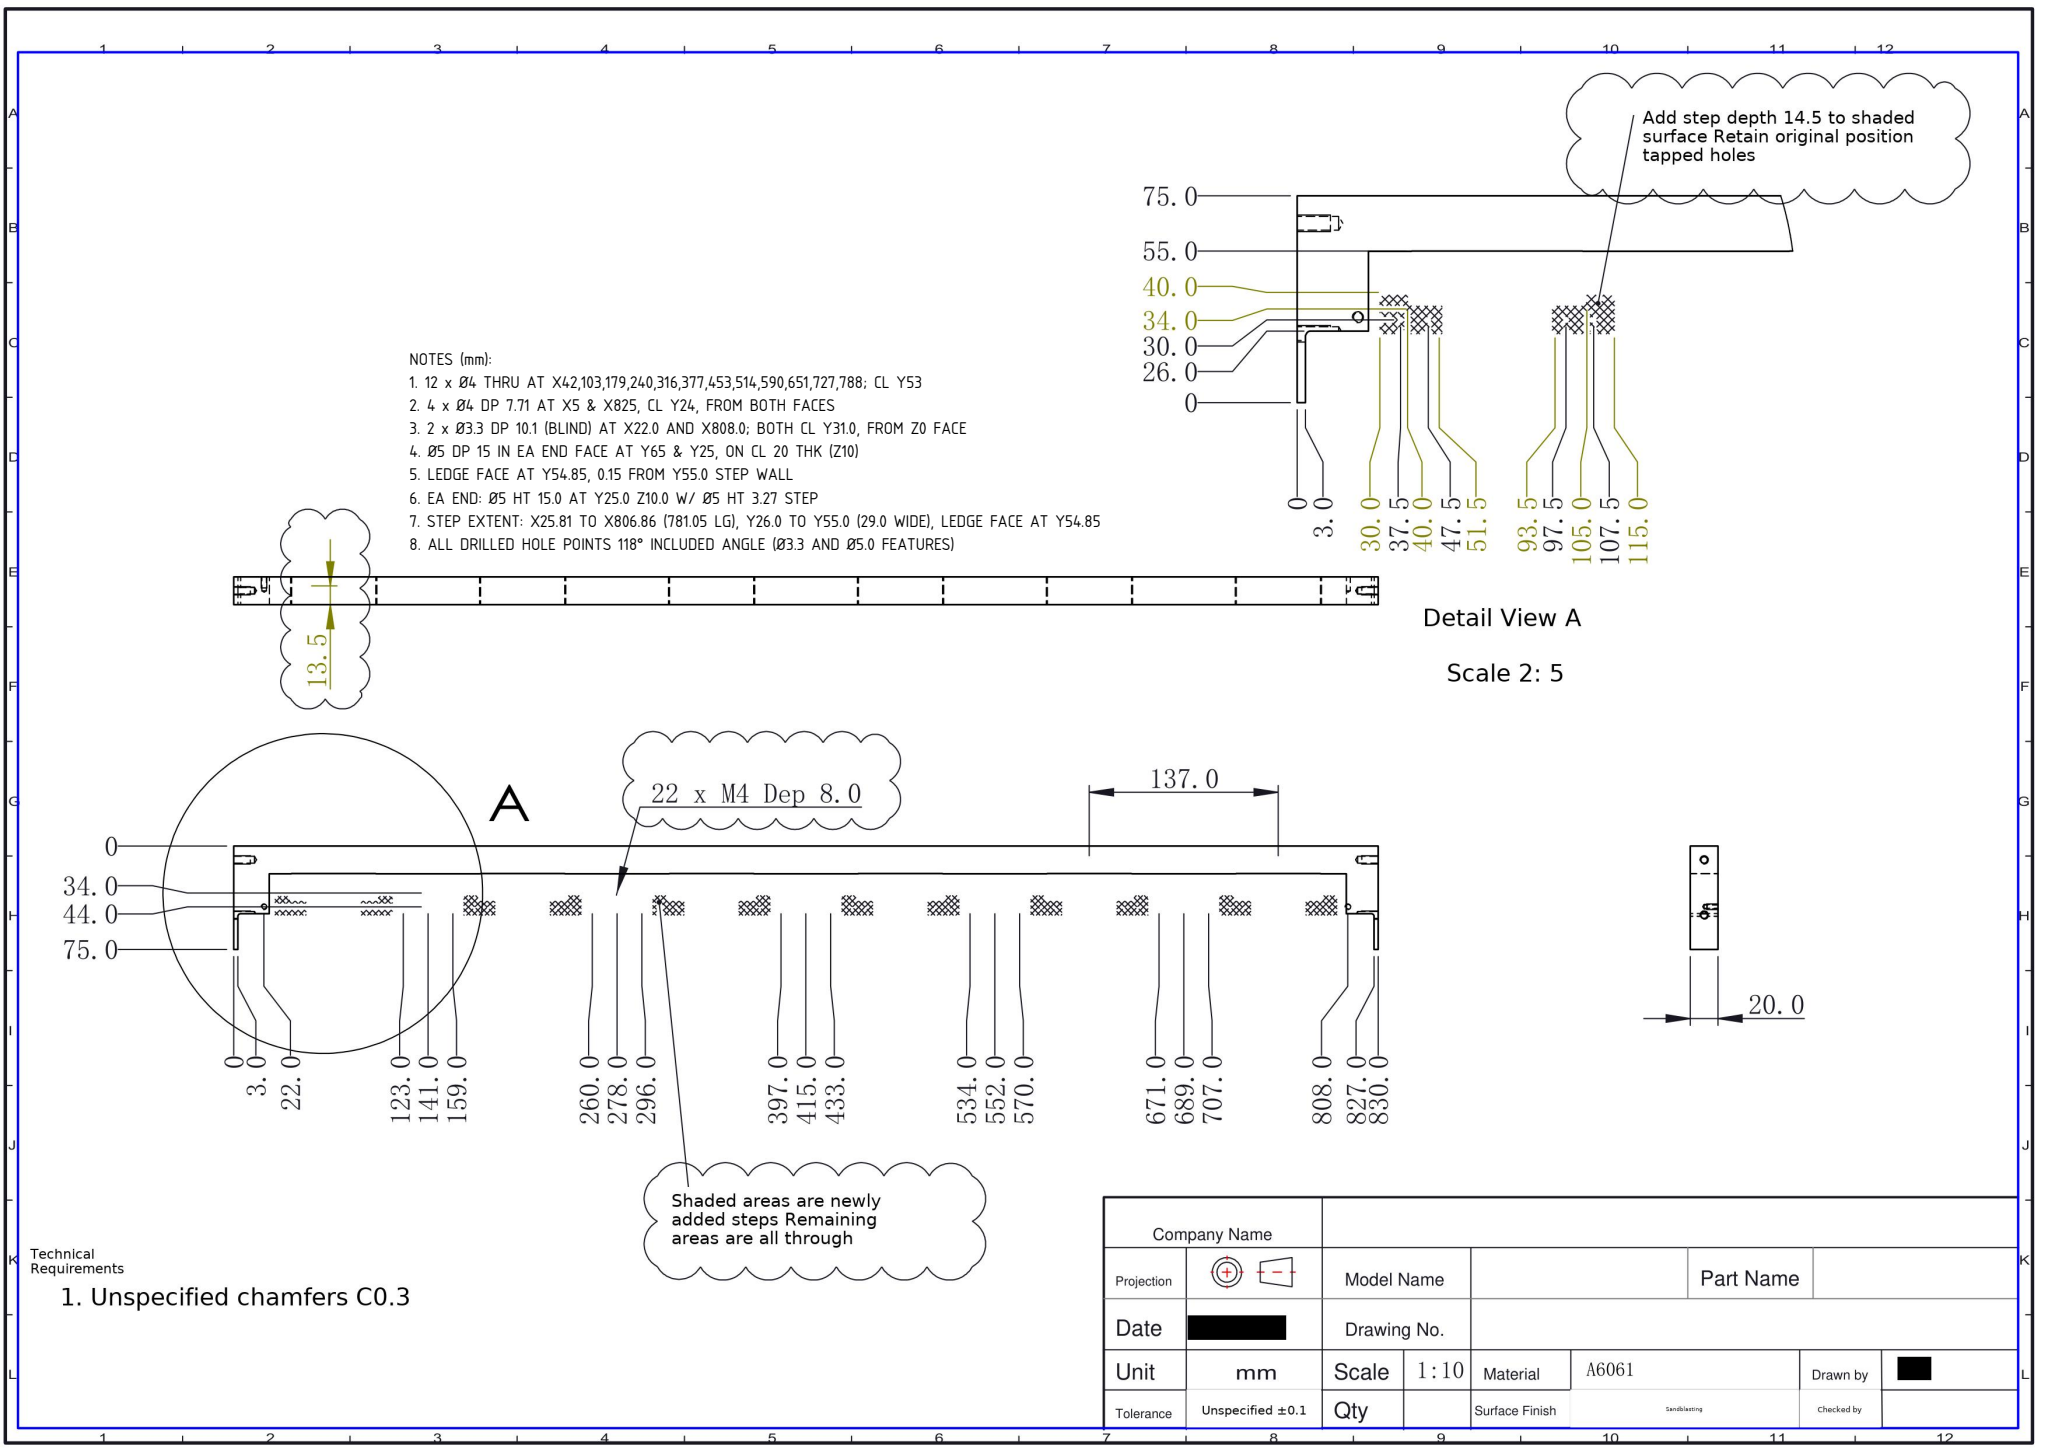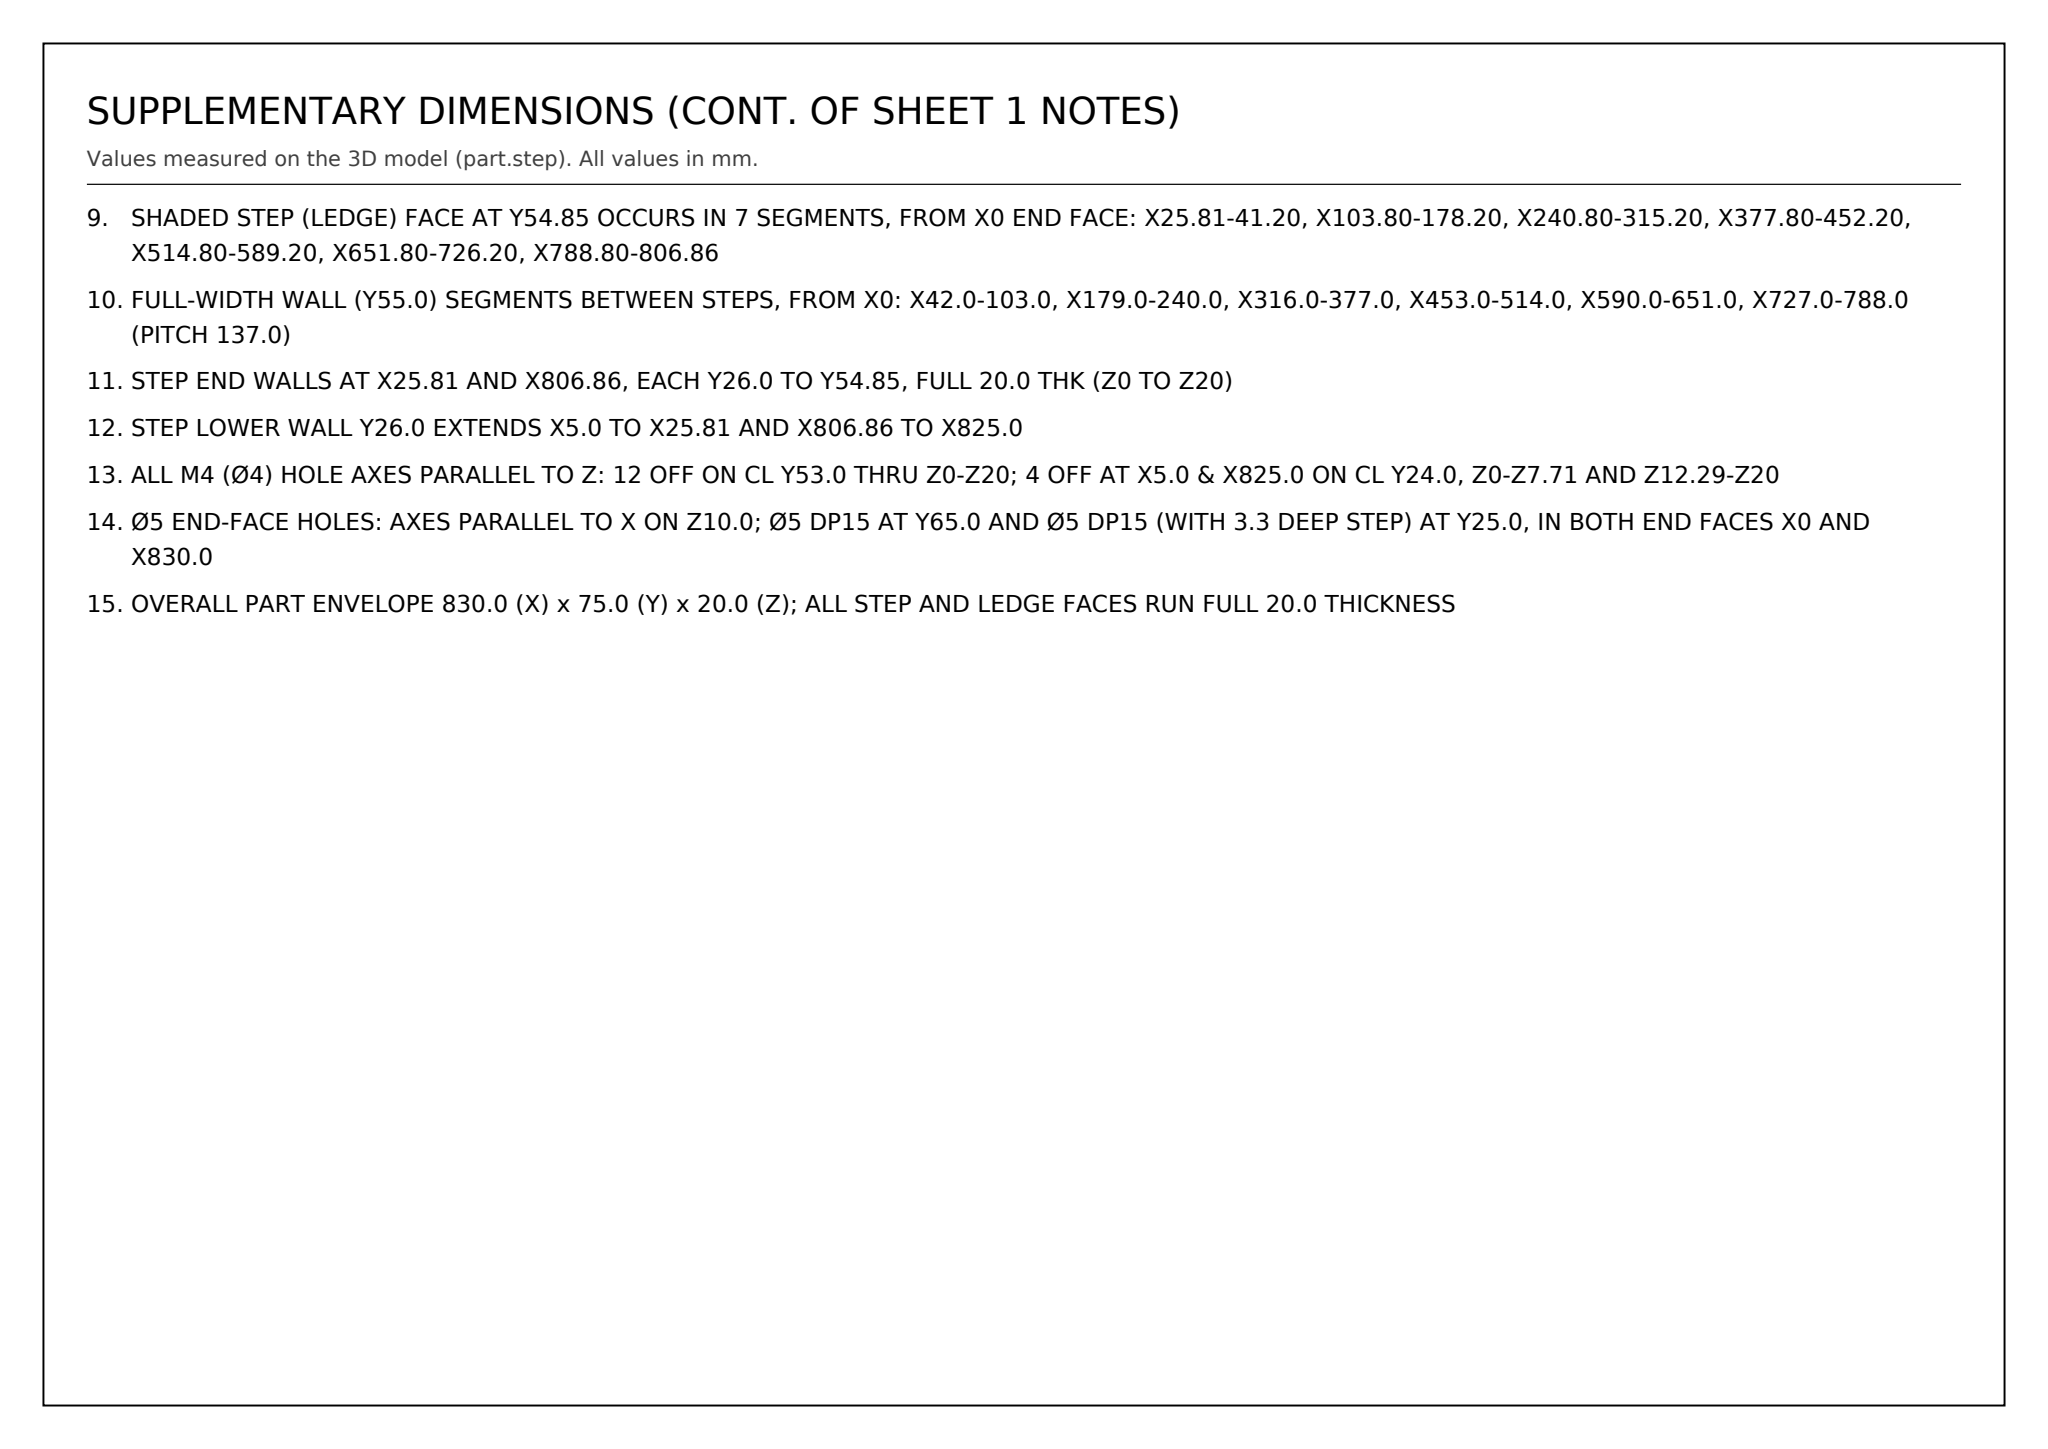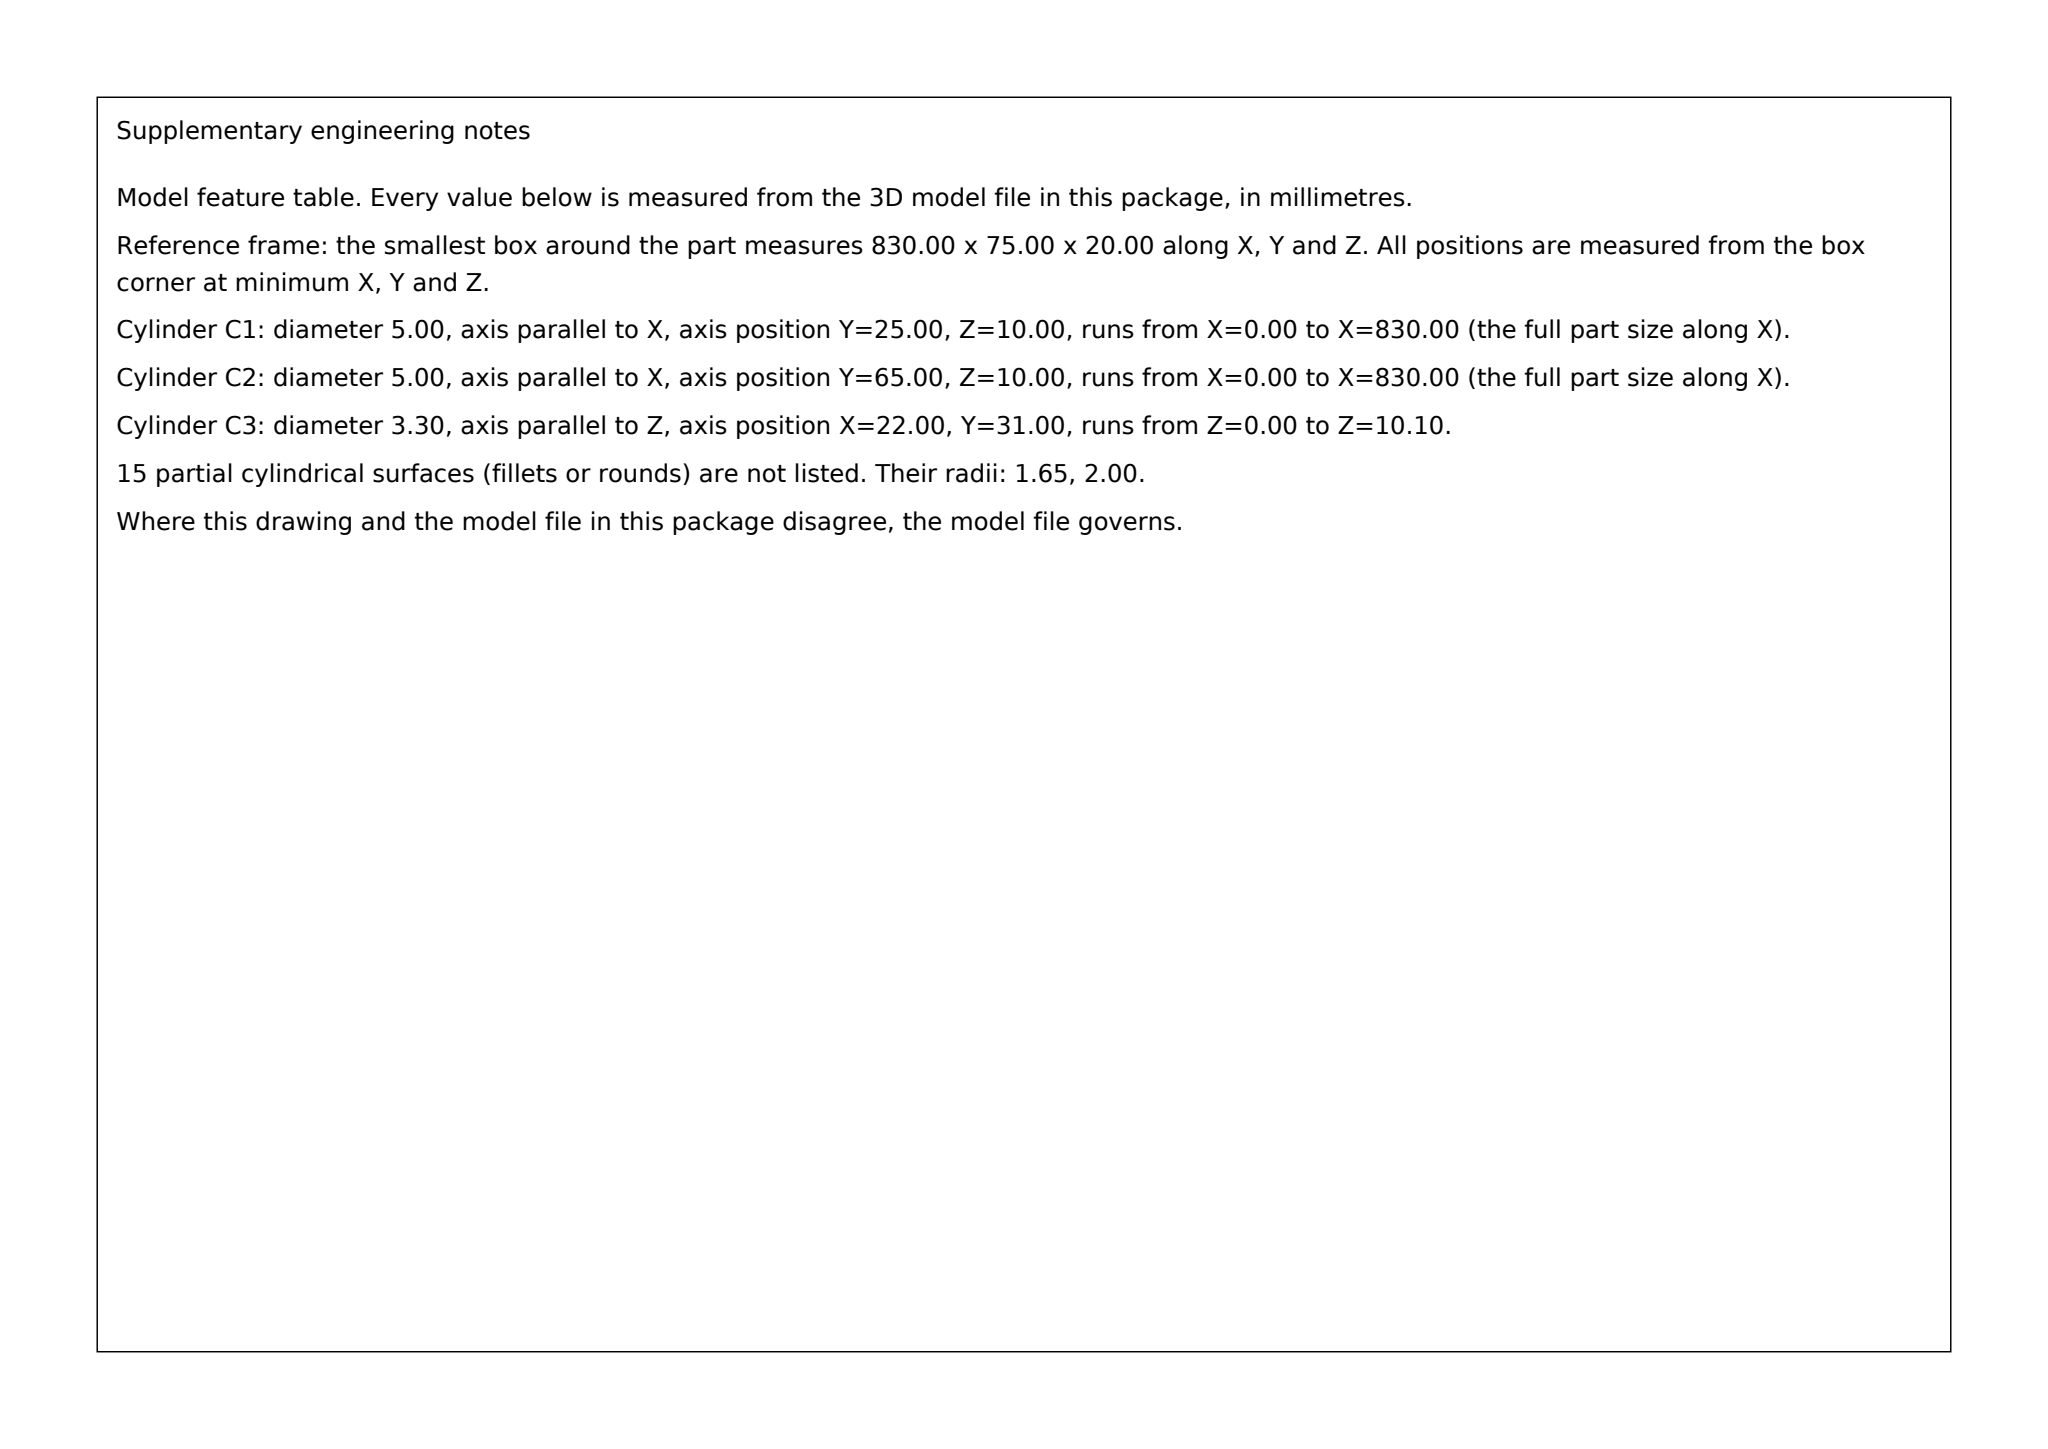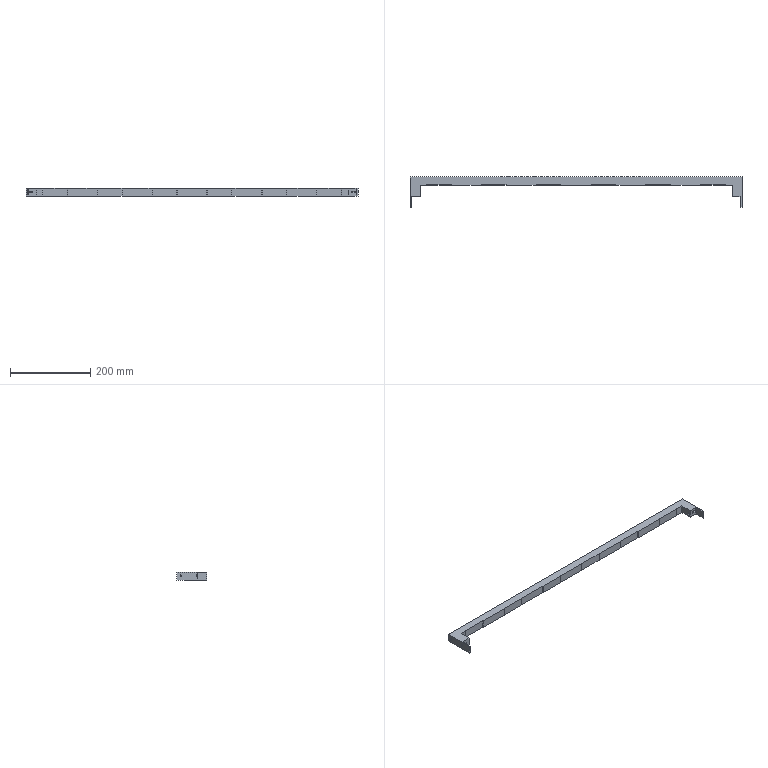Part | SolidWorks | mm | 1 solid | 63 faces | box 830 x 75 x 20 mm | volume 363775 mm3 | cylinder 27 | plane 26 | cone 10 | commonest cylinder face diameters 4 x16 5 x8 3.3 x3
Drawing notes:
12 x Ø4 THRU AT X42,103,179,240,316,377,453,514,590,651,727,788; CL Y53 | from the solid: Ø4.0 z-axis cyls L=20.0 (= full 20 thk) at y=53.0, those 12 X positions
4 x Ø4 DP 7.71 AT X5 & X825, CL Y24, FROM BOTH FACES | from the solid: Ø4.0 z-axis cyls L=7.71, count 2 each at [5,24] and [825,24]; 7.71+7.71<20 thk
2 x Ø3.3 DP 10.1 (BLIND) AT X22.0 AND X808.0; BOTH CL Y31.0, FROM Z0 FACE | from the solid: cylinders: hole/bore Ø3.3 axis z at [22.0, 31.0] from 0.0 to 10.1 (360°); Ø3.3 axis z at [808.0, 31.0] from 0.0 to 10.1 (267° arc); 118° drill-point cones at z=10.1 (bbox_from [20.4,31.0,10.1] and [806.4,31.0,10.1]); part thickness z 0-20 so holes are not through
Ø5 DP 15 IN EA END FACE AT Y65 & Y25, ON CL 20 THK (Z10) | from the solid: Ø5 x-axis cyls L=15 at [y65,z10] x4 and [y25,z10] x2; 75-65=10 from top, z10=mid-thk
LEDGE FACE AT Y54.85, 0.15 FROM Y55.0 STEP WALL | from the solid: axis_planes y=54.85 (7 faces) adjacent to y=55.0 (6 faces)
EA END: Ø5 HT 15.0 AT Y25.0 Z10.0 W/ Ø5 HT 3.27 STEP | from the solid: x-axis cyls dia 5.0 at [y25.0,z10.0]: len 15.0 count 2 and len 3.27 count 2 (one each end)
STEP EXTENT: X25.81 TO X806.86 (781.05 LG), Y26.0 TO Y55.0 (29.0 WIDE), LEDGE FACE AT Y54.85 | from the solid: axis planes x=25.81, x=806.86; y=26.0, y=54.85, y=55.0
ALL DRILLED HOLE POINTS 118° INCLUDED ANGLE (Ø3.3 AND Ø5.0 FEATURES) | from the solid: cones [118.0, 3.3, 4] and [118.0, 5.0, 6]
SHADED STEP (LEDGE) FACE AT Y54.85 OCCURS IN 7 SEGMENTS, FROM X0 END FACE: X25.81-41.20, X103.80-178.20, X240.80-315.20, X377.80-452.20, X514.80-589.20, X651.80-726.20, X788.80-806.86 | from the solid: axis_planes normal y, offset 54.8, x-extents [25.8,41.2],[103.8,178.2],[240.8,315.2],[377.8,452.2],[514.8,589.2],[651.8,726.2],[788.8,806.9]
FULL-WIDTH WALL (Y55.0) SEGMENTS BETWEEN STEPS, FROM X0: X42.0-103.0, X179.0-240.0, X316.0-377.0, X453.0-514.0, X590.0-651.0, X727.0-788.0 (PITCH 137.0) | from the solid: axis_planes normal y, offset 55.0, x-extents [42,103],[179,240],[316,377],[453,514],[590,651],[727,788]
STEP END WALLS AT X25.81 AND X806.86, EACH Y26.0 TO Y54.85, FULL 20.0 THK (Z0 TO Z20) | from the solid: axis_planes normal x at 25.8 and 806.9, extents y[26.0,54.8] z[0,20]
STEP LOWER WALL Y26.0 EXTENDS X5.0 TO X25.81 AND X806.86 TO X825.0 | from the solid: axis_planes normal y, offset 26.0, x-extents [5.0,25.8] and [806.9,825.0]
ALL M4 (Ø4) HOLE AXES PARALLEL TO Z: 12 OFF ON CL Y53.0 THRU Z0-Z20; 4 OFF AT X5.0 & X825.0 ON CL Y24.0, Z0-Z7.71 AND Z12.29-Z20 | from the solid: cylinders dia 4.0 axis z at (X,53.0) from 0.0 to 20.0; dia 4.0 axis z at (5.0,24.0) and (825.0,24.0) from 0.0-7.7 and 12.3-20.0
Ø5 END-FACE HOLES: AXES PARALLEL TO X ON Z10.0; Ø5 DP15 AT Y65.0 AND Ø5 DP15 (WITH 3.3 DEEP STEP) AT Y25.0, IN BOTH END FACES X0 AND X830.0 | from the solid: cylinders dia 5.0 axis x at (y65.0,z10.0) from 0-15 and 815-830; dia 5.0 axis x at (y25.0,z10.0) from 0-15/0-3.3 and 815-830/826.7-830
OVERALL PART ENVELOPE 830.0 (X) x 75.0 (Y) x 20.0 (Z); ALL STEP AND LEDGE FACES RUN FULL 20.0 THICKNESS | from the solid: bbox_xyz 830.001 x 75.001 x 20.001; axis_planes z at 0.0 and 20.0 spanning x[0,830] y[0,75]